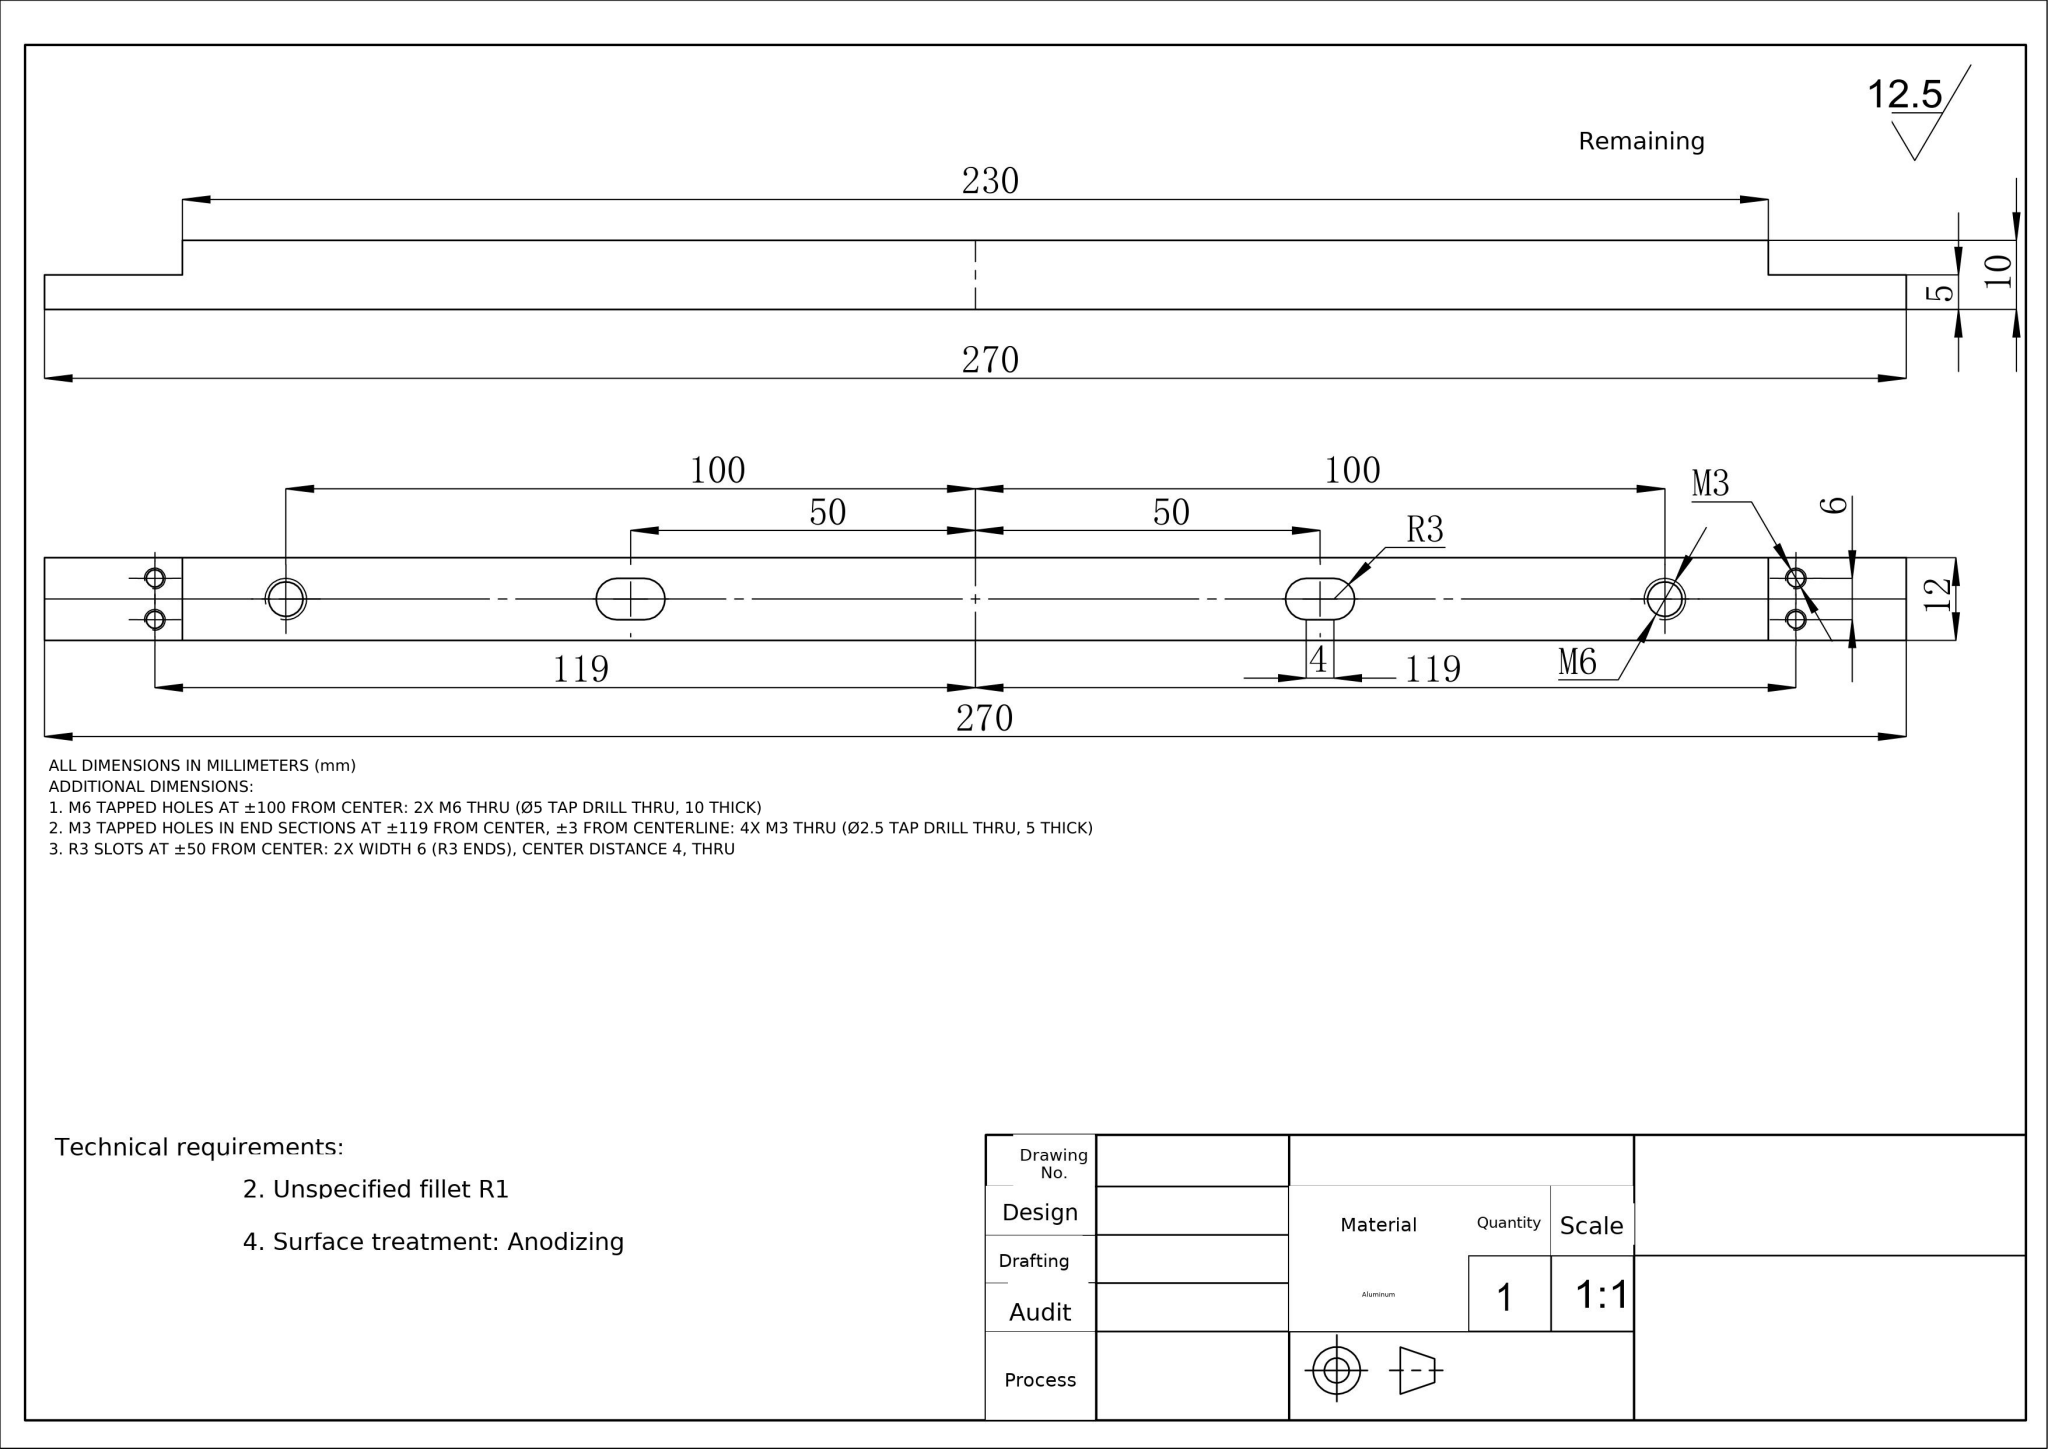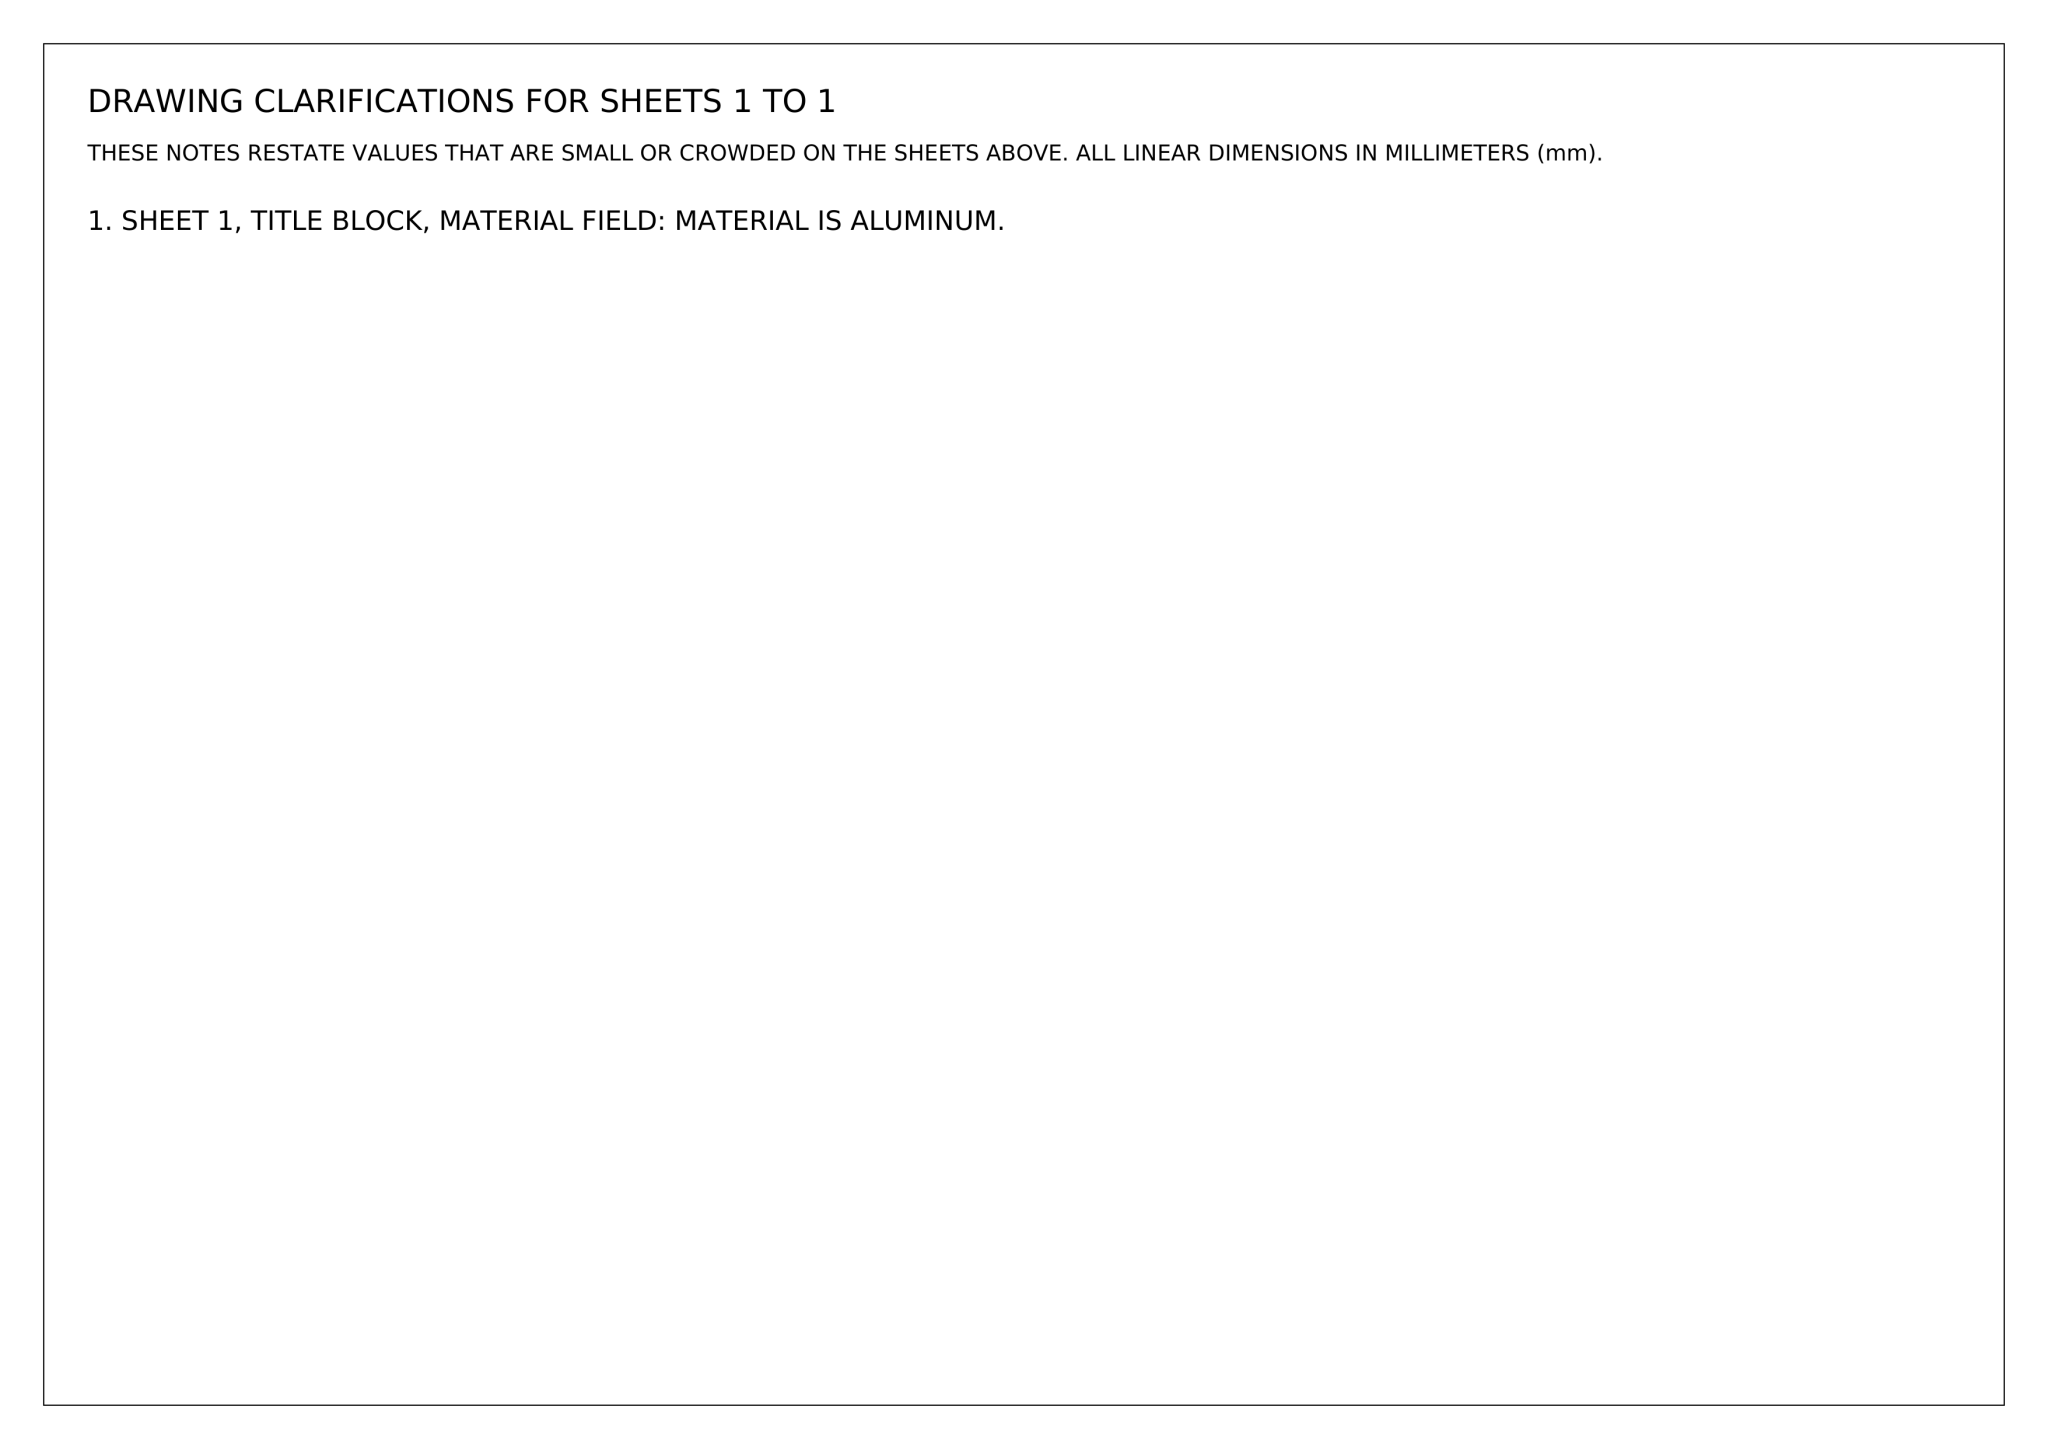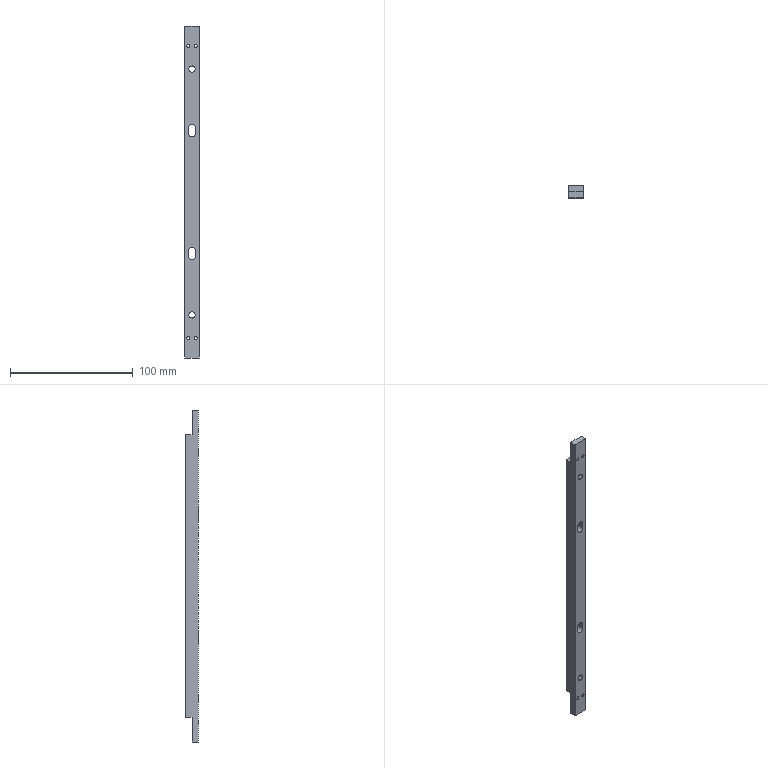Part | NX | mm | 1 solid | 32 faces | box 12 x 10 x 270 mm | volume 28464 mm3 | cylinder 18 | plane 14 | commonest cylinder face diameters 2.5 x8 6 x6 5 x4